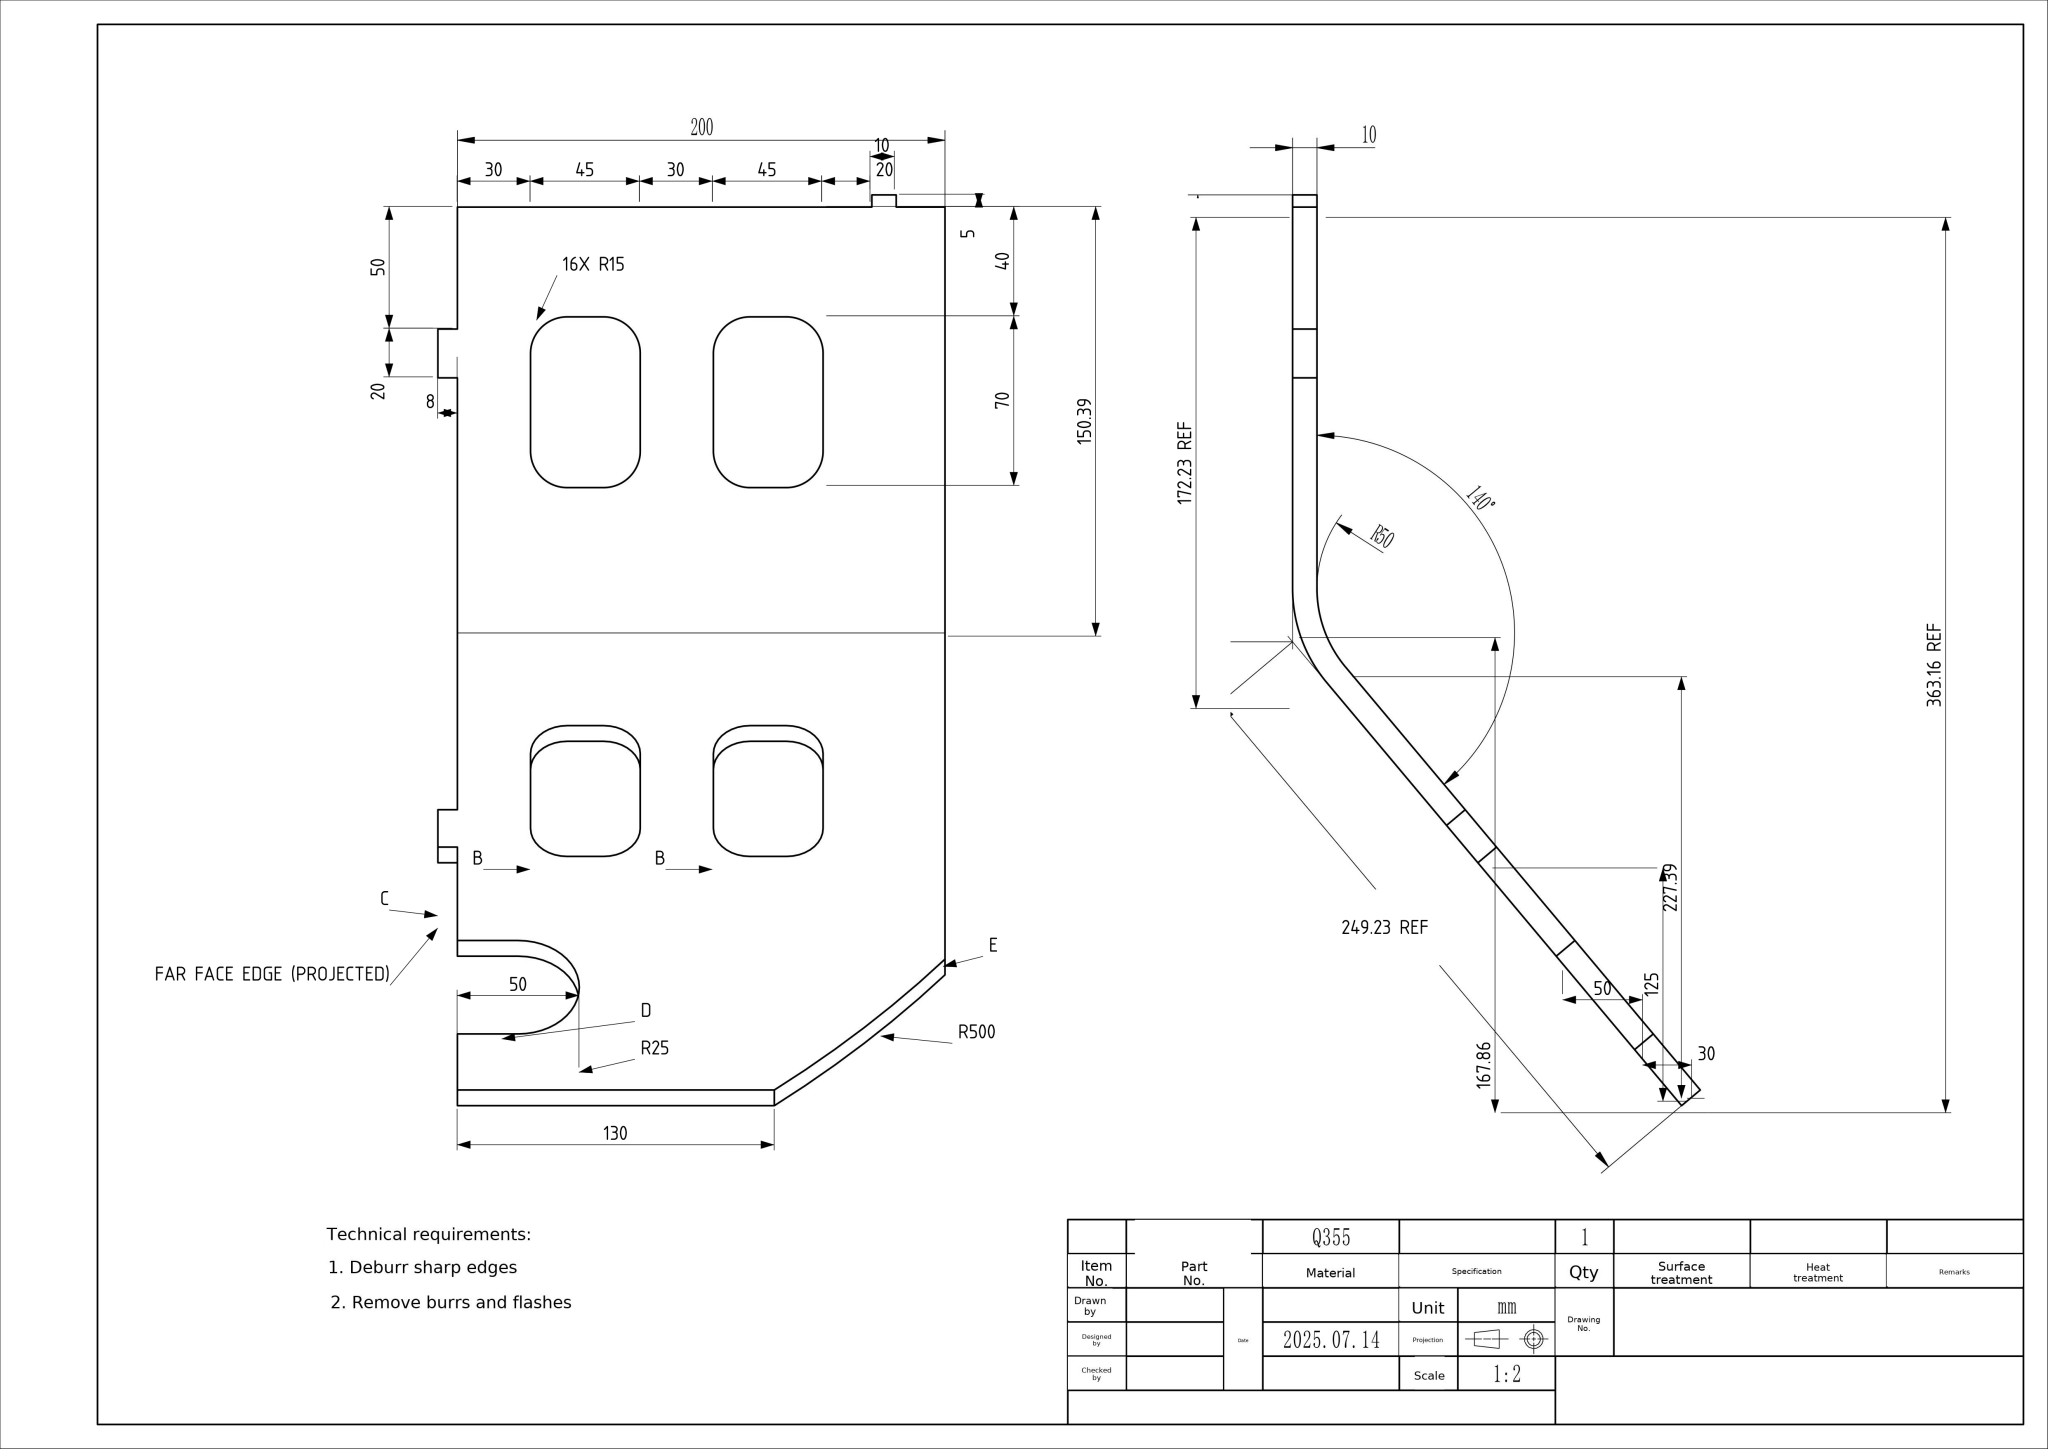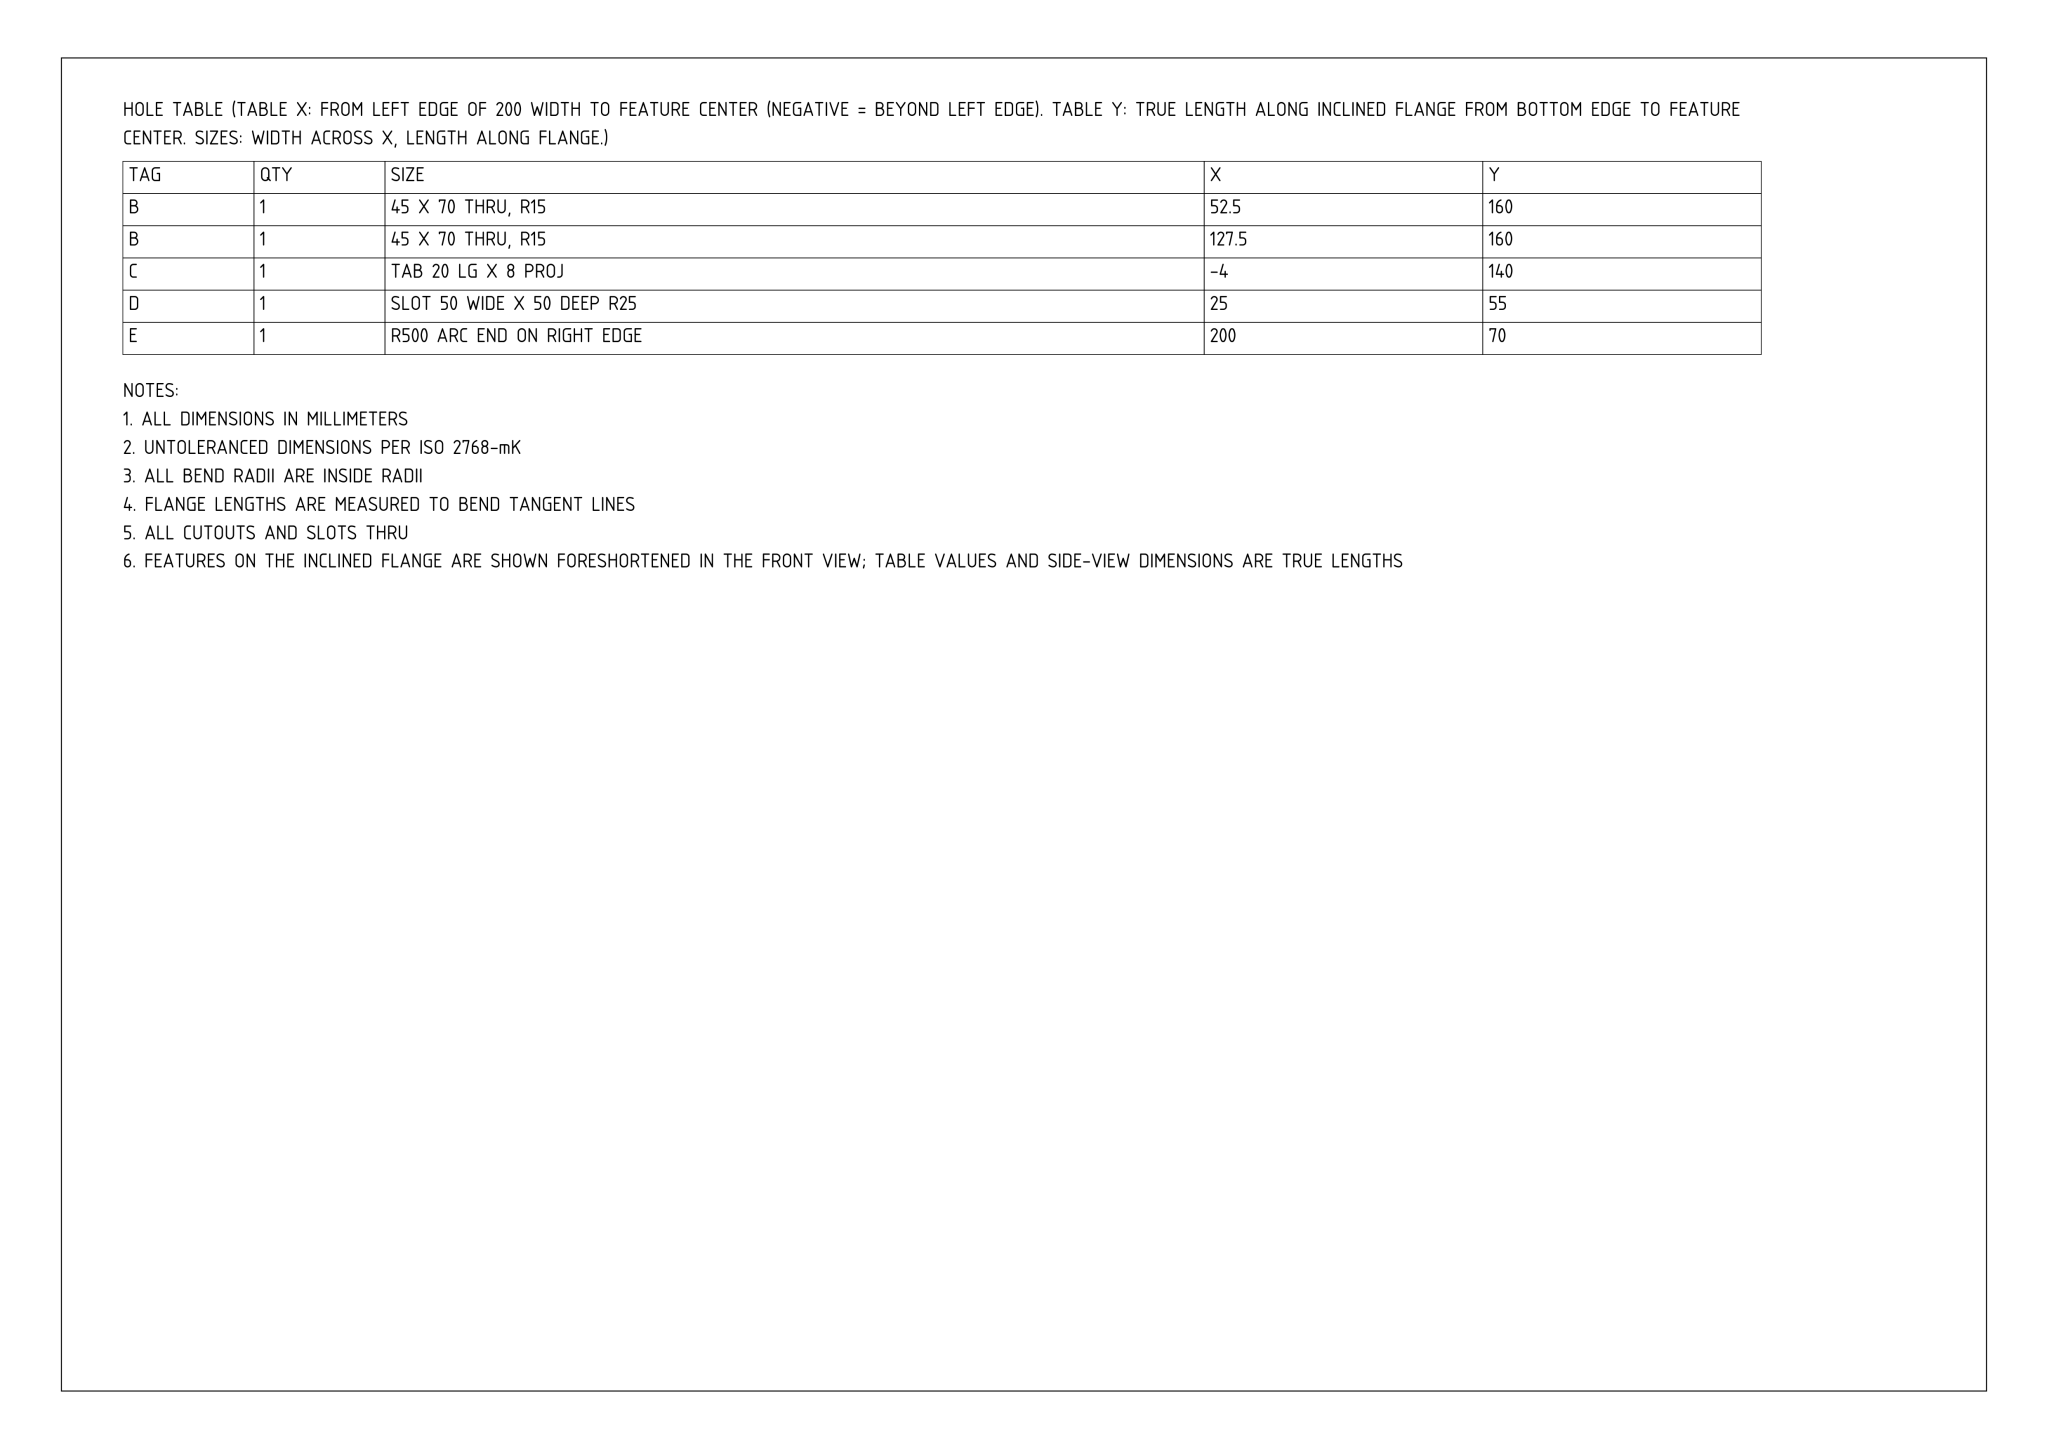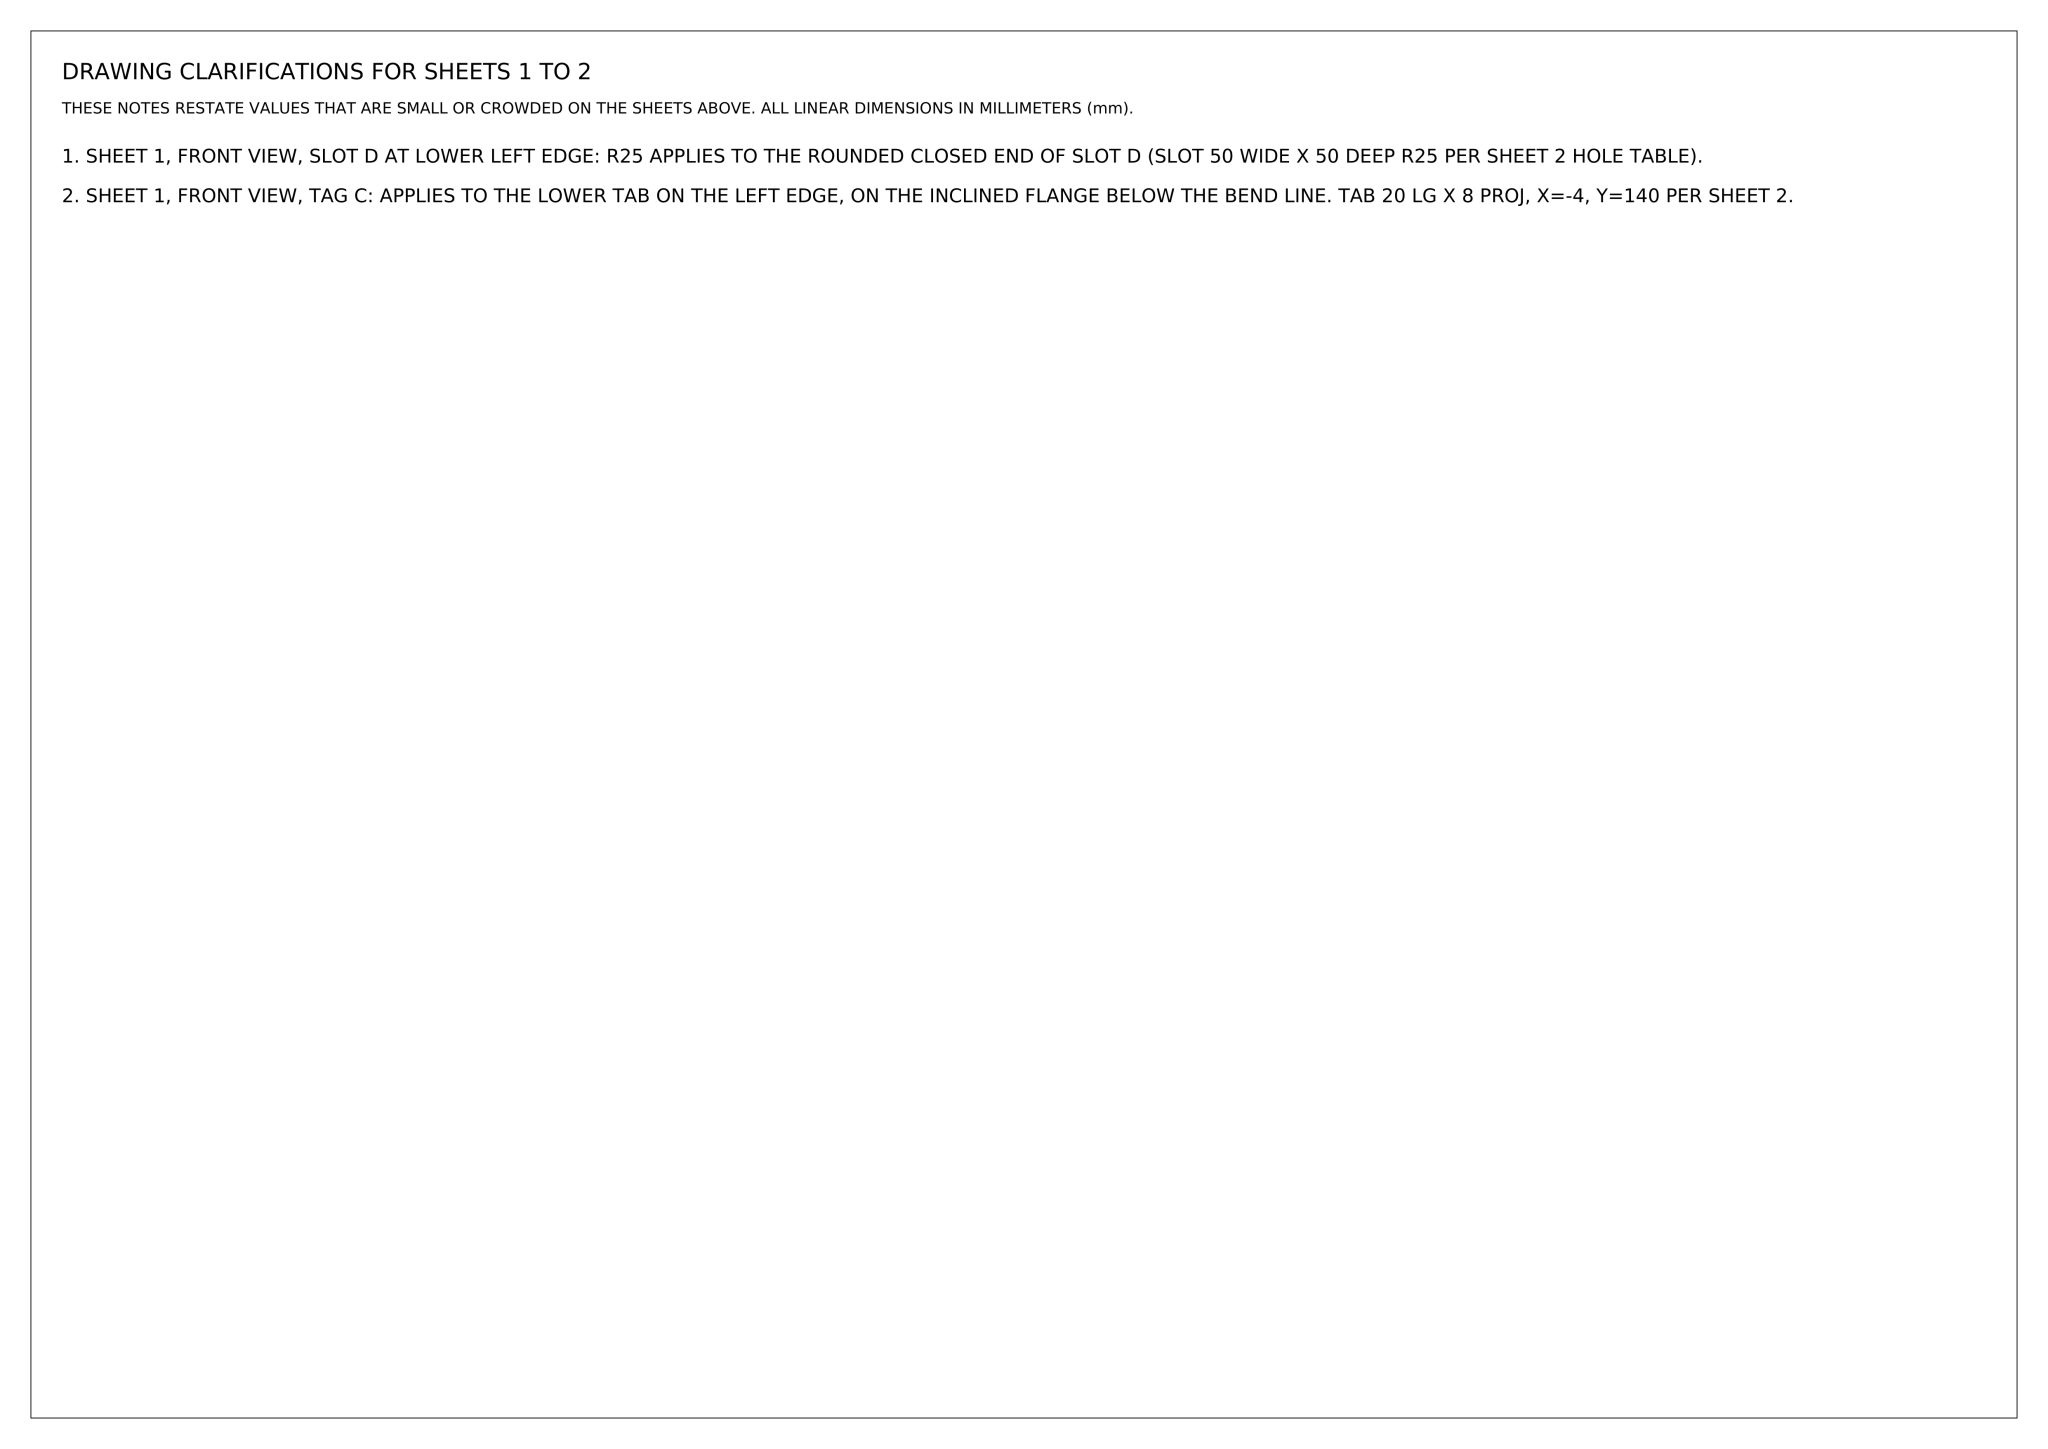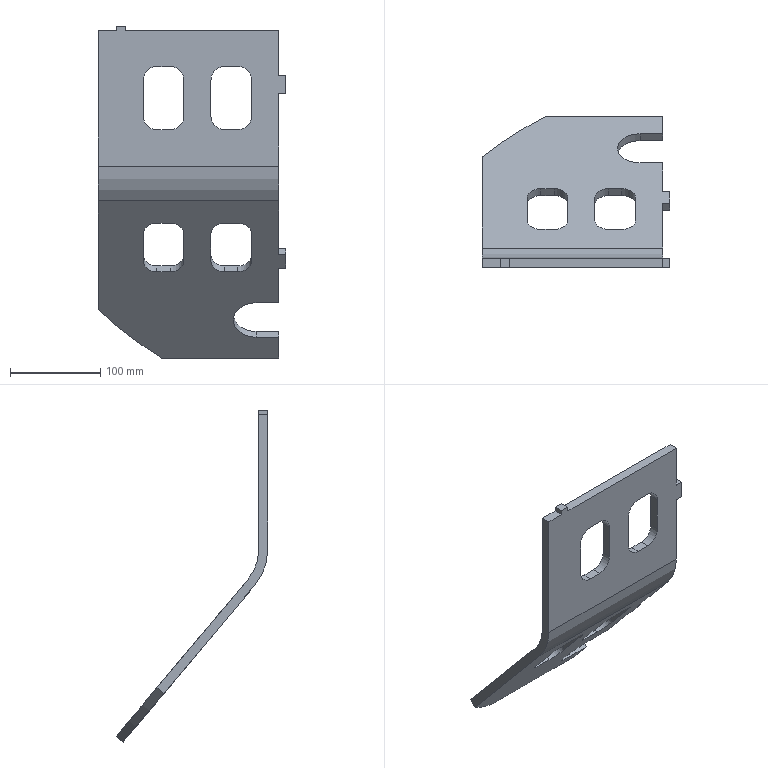Part | NX | mm | 1 solid | 59 faces | box 208 x 167.86 x 368.16 mm | volume 672604 mm3 | plane 39 | cylinder 20 | commonest cylinder face diameters 30 x16 50 x1 1000 x1 120 x1 100 x1